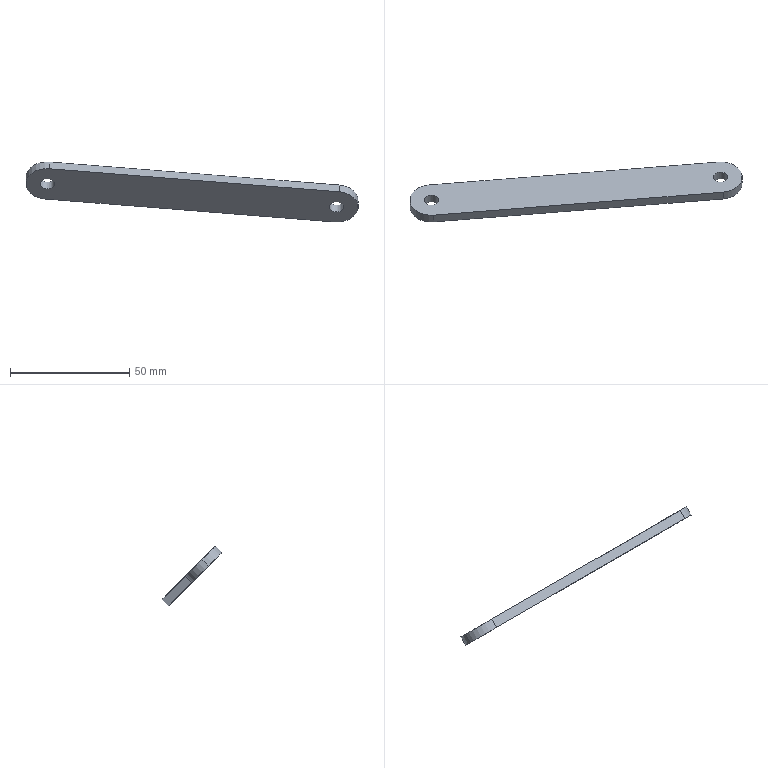Component | SolidWorks | GeneralAssembly-1_TieRod1-1 | 1 solid | 12 faces | box 139.23 x 25.21 x 25.21 mm | volume 9576 mm3 | cylinder 8 | plane 4 | commonest cylinder face diameters 6 x4 18 x4
STEP:
#1=COLOUR_RGB('',0.7922,0.8196,0.9333);
#2=FILL_AREA_STYLE_COLOUR('',#1);
#3=FILL_AREA_STYLE('',(#2));
#4=SURFACE_STYLE_FILL_AREA(#3);
#5=SURFACE_SIDE_STYLE('',(#4));
#6=SURFACE_STYLE_USAGE(.BOTH.,#5);
#7=PRESENTATION_STYLE_ASSIGNMENT((#6));
#8=CARTESIAN_POINT('',(1.617,15.691,-21.06));
#9=VERTEX_POINT('',#8);
#10=CARTESIAN_POINT('',(1.382,15.672,-21.042));
#11=VERTEX_POINT('',#10);
#12=CARTESIAN_POINT('',(1.5,15.682,-21.051));
#13=DIRECTION('',(0.,-0.7071,-0.7071));
#14=DIRECTION('',(-0.9937,-0.07912,0.07912));
#15=AXIS2_PLACEMENT_3D('',#12,#13,#14);
#16=CIRCLE('',#15,0.1181);
#17=EDGE_CURVE('',#9,#11,#16,.T.);
#18=ORIENTED_EDGE('',*,*,#17,.F.);
#19=CARTESIAN_POINT('',(1.617,15.58,-21.172));
#20=VERTEX_POINT('',#19);
#21=CARTESIAN_POINT('',(1.617,15.719,-21.032));
#22=DIRECTION('',(0.,-0.7071,-0.7071));
#23=VECTOR('',#22,39.37);
#24=LINE('',#21,#23);
#25=EDGE_CURVE('',#9,#20,#24,.T.);
#26=ORIENTED_EDGE('',*,*,#25,.T.);
#27=CARTESIAN_POINT('',(1.382,15.561,-21.153));
#28=VERTEX_POINT('',#27);
#29=CARTESIAN_POINT('',(1.5,15.57,-21.162));
#30=DIRECTION('',(0.,-0.7071,-0.7071));
#31=DIRECTION('',(-0.9937,-0.07912,0.07912));
#32=AXIS2_PLACEMENT_3D('',#29,#30,#31);
#33=CIRCLE('',#32,0.1181);
#34=EDGE_CURVE('',#20,#28,#33,.T.);
#35=ORIENTED_EDGE('',*,*,#34,.T.);
#36=CARTESIAN_POINT('',(1.382,15.7,-21.014));
#37=DIRECTION('',(0.,-0.7071,-0.7071));
#38=VECTOR('',#37,39.37);
#39=LINE('',#36,#38);
#40=EDGE_CURVE('',#11,#28,#39,.T.);
#41=ORIENTED_EDGE('',*,*,#40,.F.);
#42=EDGE_LOOP('',(#18,#26,#35,#41));
#43=FACE_OUTER_BOUND('',#42,.T.);
#44=CARTESIAN_POINT('',(1.5,15.709,-21.023));
#45=DIRECTION('',(0.,-0.7071,-0.7071));
#46=DIRECTION('',(-0.9937,-0.07912,0.07912));
#47=AXIS2_PLACEMENT_3D('',#44,#45,#46);
#48=CYLINDRICAL_SURFACE('',#47,0.1181);
#49=ADVANCED_FACE('',(#43),#48,.F.);
#50=CARTESIAN_POINT('',(6.39,16.071,-21.44));
#51=VERTEX_POINT('',#50);
#52=CARTESIAN_POINT('',(6.155,16.052,-21.422));
#53=VERTEX_POINT('',#52);
#54=CARTESIAN_POINT('',(6.273,16.062,-21.431));
#55=DIRECTION('',(0.,-0.7071,-0.7071));
#56=DIRECTION('',(-0.9937,-0.07912,0.07912));
#57=AXIS2_PLACEMENT_3D('',#54,#55,#56);
#58=CIRCLE('',#57,0.1181);
#59=EDGE_CURVE('',#51,#53,#58,.T.);
#60=ORIENTED_EDGE('',*,*,#59,.F.);
#61=CARTESIAN_POINT('',(6.39,15.96,-21.552));
#62=VERTEX_POINT('',#61);
#63=CARTESIAN_POINT('',(6.39,16.099,-21.412));
#64=DIRECTION('',(0.,-0.7071,-0.7071));
#65=VECTOR('',#64,39.37);
#66=LINE('',#63,#65);
#67=EDGE_CURVE('',#51,#62,#66,.T.);
#68=ORIENTED_EDGE('',*,*,#67,.T.);
#69=CARTESIAN_POINT('',(6.155,15.941,-21.533));
#70=VERTEX_POINT('',#69);
#71=CARTESIAN_POINT('',(6.273,15.95,-21.542));
#72=DIRECTION('',(0.,-0.7071,-0.7071));
#73=DIRECTION('',(-0.9937,-0.07912,0.07912));
#74=AXIS2_PLACEMENT_3D('',#71,#72,#73);
#75=CIRCLE('',#74,0.1181);
#76=EDGE_CURVE('',#62,#70,#75,.T.);
#77=ORIENTED_EDGE('',*,*,#76,.T.);
#78=CARTESIAN_POINT('',(6.155,16.08,-21.394));
#79=DIRECTION('',(0.,-0.7071,-0.7071));
#80=VECTOR('',#79,39.37);
#81=LINE('',#78,#80);
#82=EDGE_CURVE('',#53,#70,#81,.T.);
#83=ORIENTED_EDGE('',*,*,#82,.F.);
#84=EDGE_LOOP('',(#60,#68,#77,#83));
#85=FACE_OUTER_BOUND('',#84,.T.);
#86=CARTESIAN_POINT('',(6.273,16.089,-21.403));
#87=DIRECTION('',(0.,-0.7071,-0.7071));
#88=DIRECTION('',(-0.9937,-0.07912,0.07912));
#89=AXIS2_PLACEMENT_3D('',#86,#87,#88);
#90=CYLINDRICAL_SURFACE('',#89,0.1181);
#91=ADVANCED_FACE('',(#85),#90,.F.);
#92=CARTESIAN_POINT('',(6.312,15.813,-21.182));
#93=VERTEX_POINT('',#92);
#94=CARTESIAN_POINT('',(1.539,15.433,-20.802));
#95=VERTEX_POINT('',#94);
#96=CARTESIAN_POINT('',(6.664,15.841,-21.21));
#97=DIRECTION('',(-0.9937,-0.07912,0.07912));
#98=VECTOR('',#97,39.37);
#99=LINE('',#96,#98);
#100=EDGE_CURVE('',#93,#95,#99,.T.);
#101=ORIENTED_EDGE('',*,*,#100,.T.);
#102=CARTESIAN_POINT('',(1.539,15.321,-20.913));
#103=VERTEX_POINT('',#102);
#104=CARTESIAN_POINT('',(1.539,15.321,-20.913));
#105=DIRECTION('',(0.,-0.7071,-0.7071));
#106=VECTOR('',#105,39.37);
#107=LINE('',#104,#106);
#108=EDGE_CURVE('',#95,#103,#107,.T.);
#109=ORIENTED_EDGE('',*,*,#108,.T.);
#110=CARTESIAN_POINT('',(6.312,15.701,-21.293));
#111=VERTEX_POINT('',#110);
#112=CARTESIAN_POINT('',(6.664,15.729,-21.321));
#113=DIRECTION('',(-0.9937,-0.07912,0.07912));
#114=VECTOR('',#113,39.37);
#115=LINE('',#112,#114);
#116=EDGE_CURVE('',#111,#103,#115,.T.);
#117=ORIENTED_EDGE('',*,*,#116,.F.);
#118=CARTESIAN_POINT('',(6.312,15.701,-21.293));
#119=DIRECTION('',(-0.,0.7071,0.7071));
#120=VECTOR('',#119,39.37);
#121=LINE('',#118,#120);
#122=EDGE_CURVE('',#111,#93,#121,.T.);
#123=ORIENTED_EDGE('',*,*,#122,.T.);
#124=EDGE_LOOP('',(#101,#109,#117,#123));
#125=FACE_OUTER_BOUND('',#124,.T.);
#126=CARTESIAN_POINT('',(6.664,15.729,-21.321));
#127=DIRECTION('',(-0.1119,0.7027,-0.7027));
#128=DIRECTION('',(0.,-0.7071,-0.7071));
#129=AXIS2_PLACEMENT_3D('',#126,#127,#128);
#130=PLANE('',#129);
#131=ADVANCED_FACE('',(#125),#130,.F.);
#132=CARTESIAN_POINT('',(1.46,15.819,-21.411));
#133=VERTEX_POINT('',#132);
#134=CARTESIAN_POINT('',(6.233,16.199,-21.791));
#135=VERTEX_POINT('',#134);
#136=CARTESIAN_POINT('',(6.585,16.227,-21.819));
#137=DIRECTION('',(0.9937,0.07912,-0.07912));
#138=VECTOR('',#137,39.37);
#139=LINE('',#136,#138);
#140=EDGE_CURVE('',#133,#135,#139,.T.);
#141=ORIENTED_EDGE('',*,*,#140,.F.);
#142=CARTESIAN_POINT('',(1.46,15.931,-21.3));
#143=VERTEX_POINT('',#142);
#144=CARTESIAN_POINT('',(1.46,15.819,-21.411));
#145=DIRECTION('',(-0.,0.7071,0.7071));
#146=VECTOR('',#145,39.37);
#147=LINE('',#144,#146);
#148=EDGE_CURVE('',#133,#143,#147,.T.);
#149=ORIENTED_EDGE('',*,*,#148,.T.);
#150=CARTESIAN_POINT('',(6.233,16.311,-21.68));
#151=VERTEX_POINT('',#150);
#152=CARTESIAN_POINT('',(6.585,16.339,-21.708));
#153=DIRECTION('',(0.9937,0.07912,-0.07912));
#154=VECTOR('',#153,39.37);
#155=LINE('',#152,#154);
#156=EDGE_CURVE('',#143,#151,#155,.T.);
#157=ORIENTED_EDGE('',*,*,#156,.T.);
#158=CARTESIAN_POINT('',(6.233,16.199,-21.791));
#159=DIRECTION('',(0.,-0.7071,-0.7071));
#160=VECTOR('',#159,39.37);
#161=LINE('',#158,#160);
#162=EDGE_CURVE('',#151,#135,#161,.T.);
#163=ORIENTED_EDGE('',*,*,#162,.T.);
#164=EDGE_LOOP('',(#141,#149,#157,#163));
#165=FACE_OUTER_BOUND('',#164,.T.);
#166=CARTESIAN_POINT('',(6.585,16.227,-21.819));
#167=DIRECTION('',(0.1119,-0.7027,0.7027));
#168=DIRECTION('',(-0.,0.7071,0.7071));
#169=AXIS2_PLACEMENT_3D('',#166,#167,#168);
#170=PLANE('',#169);
#171=ADVANCED_FACE('',(#165),#170,.F.);
#172=CARTESIAN_POINT('',(1.5,15.57,-21.162));
#173=DIRECTION('',(0.,-0.7071,-0.7071));
#174=DIRECTION('',(-0.9937,-0.07912,0.07912));
#175=AXIS2_PLACEMENT_3D('',#172,#173,#174);
#176=CIRCLE('',#175,0.1181);
#177=EDGE_CURVE('',#28,#20,#176,.T.);
#178=ORIENTED_EDGE('',*,*,#177,.F.);
#179=ORIENTED_EDGE('',*,*,#34,.F.);
#180=EDGE_LOOP('',(#178,#179));
#181=FACE_BOUND('',#180,.T.);
#182=CARTESIAN_POINT('',(6.273,15.95,-21.542));
#183=DIRECTION('',(0.,-0.7071,-0.7071));
#184=DIRECTION('',(-0.9937,-0.07912,0.07912));
#185=AXIS2_PLACEMENT_3D('',#182,#183,#184);
#186=CIRCLE('',#185,0.1181);
#187=EDGE_CURVE('',#70,#62,#186,.T.);
#188=ORIENTED_EDGE('',*,*,#187,.F.);
#189=ORIENTED_EDGE('',*,*,#76,.F.);
#190=EDGE_LOOP('',(#188,#189));
#191=FACE_BOUND('',#190,.T.);
#192=CARTESIAN_POINT('',(1.148,15.542,-21.134));
#193=VERTEX_POINT('',#192);
#194=CARTESIAN_POINT('',(1.5,15.57,-21.162));
#195=DIRECTION('',(0.,-0.7071,-0.7071));
#196=DIRECTION('',(-0.9937,-0.07912,0.07912));
#197=AXIS2_PLACEMENT_3D('',#194,#195,#196);
#198=CIRCLE('',#197,0.3543);
#199=EDGE_CURVE('',#103,#193,#198,.T.);
#200=ORIENTED_EDGE('',*,*,#199,.T.);
#201=CARTESIAN_POINT('',(1.5,15.57,-21.162));
#202=DIRECTION('',(0.,-0.7071,-0.7071));
#203=DIRECTION('',(-0.9937,-0.07912,0.07912));
#204=AXIS2_PLACEMENT_3D('',#201,#202,#203);
#205=CIRCLE('',#204,0.3543);
#206=EDGE_CURVE('',#193,#133,#205,.T.);
#207=ORIENTED_EDGE('',*,*,#206,.T.);
#208=ORIENTED_EDGE('',*,*,#140,.T.);
#209=CARTESIAN_POINT('',(6.625,15.978,-21.57));
#210=VERTEX_POINT('',#209);
#211=CARTESIAN_POINT('',(6.273,15.95,-21.542));
#212=DIRECTION('',(0.,-0.7071,-0.7071));
#213=DIRECTION('',(-0.9937,-0.07912,0.07912));
#214=AXIS2_PLACEMENT_3D('',#211,#212,#213);
#215=CIRCLE('',#214,0.3543);
#216=EDGE_CURVE('',#135,#210,#215,.T.);
#217=ORIENTED_EDGE('',*,*,#216,.T.);
#218=CARTESIAN_POINT('',(6.273,15.95,-21.542));
#219=DIRECTION('',(0.,-0.7071,-0.7071));
#220=DIRECTION('',(-0.9937,-0.07912,0.07912));
#221=AXIS2_PLACEMENT_3D('',#218,#219,#220);
#222=CIRCLE('',#221,0.3543);
#223=EDGE_CURVE('',#210,#111,#222,.T.);
#224=ORIENTED_EDGE('',*,*,#223,.T.);
#225=ORIENTED_EDGE('',*,*,#116,.T.);
#226=EDGE_LOOP('',(#200,#207,#208,#217,#224,#225));
#227=FACE_OUTER_BOUND('',#226,.T.);
#228=CARTESIAN_POINT('',(2.382,15.484,-21.076));
#229=DIRECTION('',(0.,-0.7071,-0.7071));
#230=DIRECTION('',(-0.9937,-0.07912,0.07912));
#231=AXIS2_PLACEMENT_3D('',#228,#229,#230);
#232=PLANE('',#231);
#233=ADVANCED_FACE('',(#181,#191,#227),#232,.T.);
#234=CARTESIAN_POINT('',(1.5,15.682,-21.051));
#235=DIRECTION('',(0.,-0.7071,-0.7071));
#236=DIRECTION('',(-0.9937,-0.07912,0.07912));
#237=AXIS2_PLACEMENT_3D('',#234,#235,#236);
#238=CIRCLE('',#237,0.1181);
#239=EDGE_CURVE('',#11,#9,#238,.T.);
#240=ORIENTED_EDGE('',*,*,#239,.T.);
#241=ORIENTED_EDGE('',*,*,#17,.T.);
#242=EDGE_LOOP('',(#240,#241));
#243=FACE_BOUND('',#242,.T.);
#244=CARTESIAN_POINT('',(6.273,16.062,-21.431));
#245=DIRECTION('',(0.,-0.7071,-0.7071));
#246=DIRECTION('',(-0.9937,-0.07912,0.07912));
#247=AXIS2_PLACEMENT_3D('',#244,#245,#246);
#248=CIRCLE('',#247,0.1181);
#249=EDGE_CURVE('',#53,#51,#248,.T.);
#250=ORIENTED_EDGE('',*,*,#249,.T.);
#251=ORIENTED_EDGE('',*,*,#59,.T.);
#252=EDGE_LOOP('',(#250,#251));
#253=FACE_BOUND('',#252,.T.);
#254=ORIENTED_EDGE('',*,*,#156,.F.);
#255=CARTESIAN_POINT('',(1.148,15.654,-21.023));
#256=VERTEX_POINT('',#255);
#257=CARTESIAN_POINT('',(1.5,15.682,-21.051));
#258=DIRECTION('',(-0.,0.7071,0.7071));
#259=DIRECTION('',(-0.9937,-0.07912,0.07912));
#260=AXIS2_PLACEMENT_3D('',#257,#258,#259);
#261=CIRCLE('',#260,0.3543);
#262=EDGE_CURVE('',#143,#256,#261,.T.);
#263=ORIENTED_EDGE('',*,*,#262,.T.);
#264=CARTESIAN_POINT('',(1.5,15.682,-21.051));
#265=DIRECTION('',(-0.,0.7071,0.7071));
#266=DIRECTION('',(-0.9937,-0.07912,0.07912));
#267=AXIS2_PLACEMENT_3D('',#264,#265,#266);
#268=CIRCLE('',#267,0.3543);
#269=EDGE_CURVE('',#256,#95,#268,.T.);
#270=ORIENTED_EDGE('',*,*,#269,.T.);
#271=ORIENTED_EDGE('',*,*,#100,.F.);
#272=CARTESIAN_POINT('',(6.625,16.09,-21.459));
#273=VERTEX_POINT('',#272);
#274=CARTESIAN_POINT('',(6.273,16.062,-21.431));
#275=DIRECTION('',(-0.,0.7071,0.7071));
#276=DIRECTION('',(-0.9937,-0.07912,0.07912));
#277=AXIS2_PLACEMENT_3D('',#274,#275,#276);
#278=CIRCLE('',#277,0.3543);
#279=EDGE_CURVE('',#93,#273,#278,.T.);
#280=ORIENTED_EDGE('',*,*,#279,.T.);
#281=CARTESIAN_POINT('',(6.273,16.062,-21.431));
#282=DIRECTION('',(-0.,0.7071,0.7071));
#283=DIRECTION('',(-0.9937,-0.07912,0.07912));
#284=AXIS2_PLACEMENT_3D('',#281,#282,#283);
#285=CIRCLE('',#284,0.3543);
#286=EDGE_CURVE('',#273,#151,#285,.T.);
#287=ORIENTED_EDGE('',*,*,#286,.T.);
#288=EDGE_LOOP('',(#254,#263,#270,#271,#280,#287));
#289=FACE_OUTER_BOUND('',#288,.T.);
#290=CARTESIAN_POINT('',(2.382,15.595,-20.965));
#291=DIRECTION('',(0.,-0.7071,-0.7071));
#292=DIRECTION('',(-0.9937,-0.07912,0.07912));
#293=AXIS2_PLACEMENT_3D('',#290,#291,#292);
#294=PLANE('',#293);
#295=ADVANCED_FACE('',(#243,#253,#289),#294,.F.);
#296=CARTESIAN_POINT('',(1.148,15.542,-21.134));
#297=DIRECTION('',(-0.,0.7071,0.7071));
#298=VECTOR('',#297,39.37);
#299=LINE('',#296,#298);
#300=EDGE_CURVE('',#193,#256,#299,.T.);
#301=ORIENTED_EDGE('',*,*,#300,.F.);
#302=ORIENTED_EDGE('',*,*,#199,.F.);
#303=ORIENTED_EDGE('',*,*,#108,.F.);
#304=ORIENTED_EDGE('',*,*,#269,.F.);
#305=EDGE_LOOP('',(#301,#302,#303,#304));
#306=FACE_OUTER_BOUND('',#305,.T.);
#307=CARTESIAN_POINT('',(1.5,15.57,-21.162));
#308=DIRECTION('',(-0.,0.7071,0.7071));
#309=DIRECTION('',(0.9937,0.07912,-0.07912));
#310=AXIS2_PLACEMENT_3D('',#307,#308,#309);
#311=CYLINDRICAL_SURFACE('',#310,0.3543);
#312=ADVANCED_FACE('',(#306),#311,.T.);
#313=ORIENTED_EDGE('',*,*,#206,.F.);
#314=ORIENTED_EDGE('',*,*,#300,.T.);
#315=ORIENTED_EDGE('',*,*,#262,.F.);
#316=ORIENTED_EDGE('',*,*,#148,.F.);
#317=EDGE_LOOP('',(#313,#314,#315,#316));
#318=FACE_OUTER_BOUND('',#317,.T.);
#319=CARTESIAN_POINT('',(1.5,15.57,-21.162));
#320=DIRECTION('',(-0.,0.7071,0.7071));
#321=DIRECTION('',(0.9937,0.07912,-0.07912));
#322=AXIS2_PLACEMENT_3D('',#319,#320,#321);
#323=CYLINDRICAL_SURFACE('',#322,0.3543);
#324=ADVANCED_FACE('',(#318),#323,.T.);
#325=ORIENTED_EDGE('',*,*,#122,.F.);
#326=ORIENTED_EDGE('',*,*,#223,.F.);
#327=CARTESIAN_POINT('',(6.625,15.978,-21.57));
#328=DIRECTION('',(0.,-0.7071,-0.7071));
#329=VECTOR('',#328,39.37);
#330=LINE('',#327,#329);
#331=EDGE_CURVE('',#273,#210,#330,.T.);
#332=ORIENTED_EDGE('',*,*,#331,.F.);
#333=ORIENTED_EDGE('',*,*,#279,.F.);
#334=EDGE_LOOP('',(#325,#326,#332,#333));
#335=FACE_OUTER_BOUND('',#334,.T.);
#336=CARTESIAN_POINT('',(6.273,15.95,-21.542));
#337=DIRECTION('',(-0.,0.7071,0.7071));
#338=DIRECTION('',(0.9937,0.07912,-0.07912));
#339=AXIS2_PLACEMENT_3D('',#336,#337,#338);
#340=CYLINDRICAL_SURFACE('',#339,0.3543);
#341=ADVANCED_FACE('',(#335),#340,.T.);
#342=ORIENTED_EDGE('',*,*,#216,.F.);
#343=ORIENTED_EDGE('',*,*,#162,.F.);
#344=ORIENTED_EDGE('',*,*,#286,.F.);
#345=ORIENTED_EDGE('',*,*,#331,.T.);
#346=EDGE_LOOP('',(#342,#343,#344,#345));
#347=FACE_OUTER_BOUND('',#346,.T.);
#348=CARTESIAN_POINT('',(6.273,15.95,-21.542));
#349=DIRECTION('',(-0.,0.7071,0.7071));
#350=DIRECTION('',(0.9937,0.07912,-0.07912));
#351=AXIS2_PLACEMENT_3D('',#348,#349,#350);
#352=CYLINDRICAL_SURFACE('',#351,0.3543);
#353=ADVANCED_FACE('',(#347),#352,.T.);
#354=ORIENTED_EDGE('',*,*,#67,.F.);
#355=ORIENTED_EDGE('',*,*,#249,.F.);
#356=ORIENTED_EDGE('',*,*,#82,.T.);
#357=ORIENTED_EDGE('',*,*,#187,.T.);
#358=EDGE_LOOP('',(#354,#355,#356,#357));
#359=FACE_OUTER_BOUND('',#358,.T.);
#360=CARTESIAN_POINT('',(6.273,16.089,-21.403));
#361=DIRECTION('',(0.,-0.7071,-0.7071));
#362=DIRECTION('',(-0.9937,-0.07912,0.07912));
#363=AXIS2_PLACEMENT_3D('',#360,#361,#362);
#364=CYLINDRICAL_SURFACE('',#363,0.1181);
#365=ADVANCED_FACE('',(#359),#364,.F.);
#366=ORIENTED_EDGE('',*,*,#25,.F.);
#367=ORIENTED_EDGE('',*,*,#239,.F.);
#368=ORIENTED_EDGE('',*,*,#40,.T.);
#369=ORIENTED_EDGE('',*,*,#177,.T.);
#370=EDGE_LOOP('',(#366,#367,#368,#369));
#371=FACE_OUTER_BOUND('',#370,.T.);
#372=CARTESIAN_POINT('',(1.5,15.709,-21.023));
#373=DIRECTION('',(0.,-0.7071,-0.7071));
#374=DIRECTION('',(-0.9937,-0.07912,0.07912));
#375=AXIS2_PLACEMENT_3D('',#372,#373,#374);
#376=CYLINDRICAL_SURFACE('',#375,0.1181);
#377=ADVANCED_FACE('',(#371),#376,.F.);
#378=CLOSED_SHELL('',(#49,#91,#131,#171,#233,#295,#312,#324,#341,#353,#365,#377));
#379=MANIFOLD_SOLID_BREP('',#378);
#380=STYLED_ITEM('',(#7),#379);
#381=(LENGTH_UNIT()NAMED_UNIT(*)SI_UNIT($,.METRE.));
#382=LENGTH_MEASURE_WITH_UNIT(LENGTH_MEASURE(0.0254),#381);
#383=DIMENSIONAL_EXPONENTS(1.,0.,0.,0.,0.,0.,0.);
#384=(CONVERSION_BASED_UNIT('',#382)LENGTH_UNIT()NAMED_UNIT(#383));
#385=UNCERTAINTY_MEASURE_WITH_UNIT(LENGTH_MEASURE(0.00001),#384,'','');
#386=(NAMED_UNIT(*)PLANE_ANGLE_UNIT()SI_UNIT($,.RADIAN.));
#387=(NAMED_UNIT(*)SI_UNIT($,.STERADIAN.)SOLID_ANGLE_UNIT());
#388=(GEOMETRIC_REPRESENTATION_CONTEXT(3)GLOBAL_UNCERTAINTY_ASSIGNED_CONTEXT((#385))GLOBAL_UNIT_ASSIGNED_CONTEXT((#384,#386,#387))REPRESENTATION_CONTEXT('',''));
#389=MECHANICAL_DESIGN_GEOMETRIC_PRESENTATION_REPRESENTATION('',(#380),#388);
#390=PRESENTATION_LAYER_ASSIGNMENT('','',(#380));
#391=CARTESIAN_POINT('',(0.,0.,0.));
#392=DIRECTION('',(0.,0.,1.));
#393=DIRECTION('',(1.,0.,0.));
#394=AXIS2_PLACEMENT_3D('',#391,#392,#393);
#395=(LENGTH_UNIT()NAMED_UNIT(*)SI_UNIT($,.METRE.));
#396=LENGTH_MEASURE_WITH_UNIT(LENGTH_MEASURE(0.0254),#395);
#397=DIMENSIONAL_EXPONENTS(1.,0.,0.,0.,0.,0.,0.);
#398=(CONVERSION_BASED_UNIT('',#396)LENGTH_UNIT()NAMED_UNIT(#397));
#399=UNCERTAINTY_MEASURE_WITH_UNIT(LENGTH_MEASURE(0.00001),#398,'','');
#400=(NAMED_UNIT(*)PLANE_ANGLE_UNIT()SI_UNIT($,.RADIAN.));
#401=(NAMED_UNIT(*)SI_UNIT($,.STERADIAN.)SOLID_ANGLE_UNIT());
#402=(GEOMETRIC_REPRESENTATION_CONTEXT(3)GLOBAL_UNCERTAINTY_ASSIGNED_CONTEXT((#399))GLOBAL_UNIT_ASSIGNED_CONTEXT((#398,#400,#401))REPRESENTATION_CONTEXT('',''));
#403=ADVANCED_BREP_SHAPE_REPRESENTATION('',(#379,#394),#402);